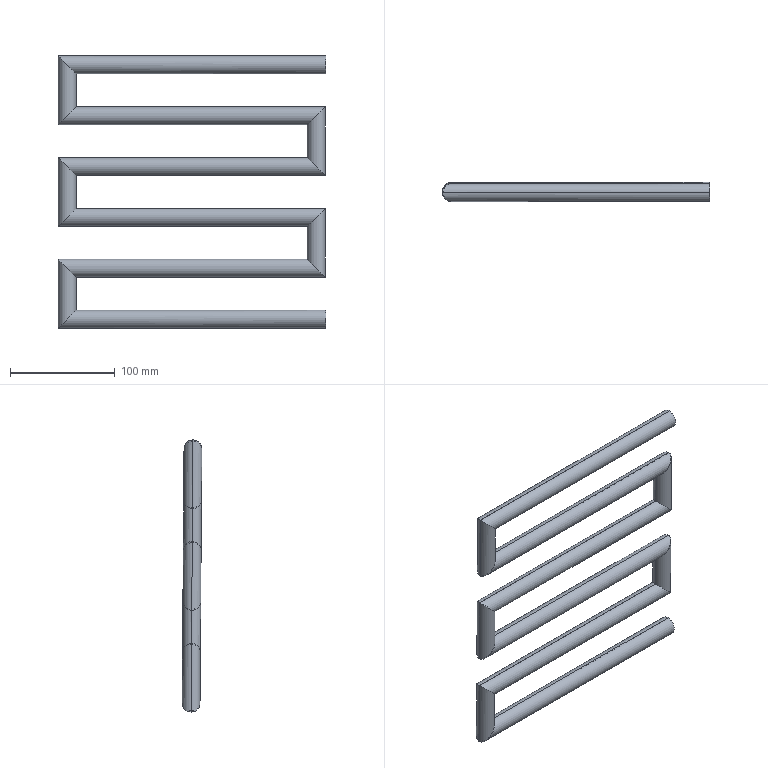Component | SolidWorks | HeatExchangePlate-1_HeatPipe-1 | 1 solid | 46 faces | box 255 x 18.76 x 259.49 mm | volume 84726 mm3 | cylinder 44 | plane 2 | commonest cylinder face diameters 15 x22 17 x22
build123d program:
from build123d import *

# Parameters (mm, degrees)
SKETCH1_R           = 8.5
SKETCH1_R_2         = 7.5
SKETCH3_R           = 8.5
SKETCH3_R_2         = 7.5
BOSS_EXTRUDE1_DEPTH = 8.98


with BuildPart() as part:
    # Sweep1: sweep along a path in Sketch2
    with BuildLine(Plane(origin=(0, 0, 0), x_dir=(1, 0, 0), z_dir=(0, 1, 0))) as sweep1_path:
        Line((0, 0), (0, 237.52))
        Line((0, 237.52), (-48.5, 237.52))
        Line((-48.5, 237.52), (-48.5, 0))
        Line((-48.5, 0), (-97, 0))
        Line((-97, 0), (-97, 237.52))
        Line((-97, 237.52), (-145.5, 237.52))
        Line((-145.5, 237.52), (-145.5, 0))
        Line((-145.5, 0), (-194, 0))
        Line((-194, 0), (-194, 237.52))
        Line((-194, 237.52), (-242.5, 237.52))
        Line((-242.5, 237.52), (-242.5, 0))
    # Sketch1 → Sweep1 (sweep)
    with BuildSketch(Plane.XY):
        Circle(SKETCH1_R)
        Circle(SKETCH1_R_2, mode=Mode.SUBTRACT)
    sweep(path=sweep1_path.line, transition=Transition.RIGHT)

    # Sketch3 → Boss-Extrude1 (add)
    # profile 1 of 2: a face of its own
    with BuildSketch(Plane.XY):
        with Locations(Location((-242.5, 0, 0), (0, 0, 180))):
            Circle(SKETCH3_R)
        with Locations(Location((-242.5, 0, 0), (0, 0, 180))):
            Circle(SKETCH3_R_2, mode=Mode.SUBTRACT)
    # profile 2 of 2: a face of its own
    with BuildSketch(Plane.XY):
        Circle(SKETCH3_R)
        Circle(SKETCH3_R_2, mode=Mode.SUBTRACT)
    extrude(amount=BOSS_EXTRUDE1_DEPTH)


solid = part.part

# Placed as in the assembly
solid = solid.moved(Location((577.41, 810.2, 125), (-179.584, 90, 0)))